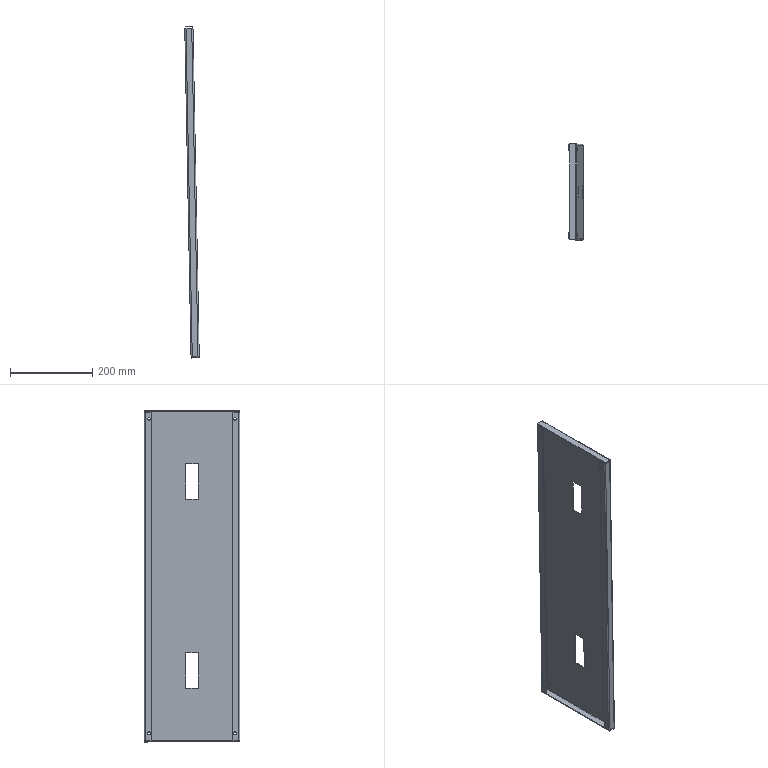Component | SolidWorks | 04FrameEndPlate3-1 | 1 solid | 88 faces | volume 479463 mm3 | plane 60 | cylinder 28 | commonest cylinder face diameters 7 x16 6 x6 2 x6 | material A3 Steel